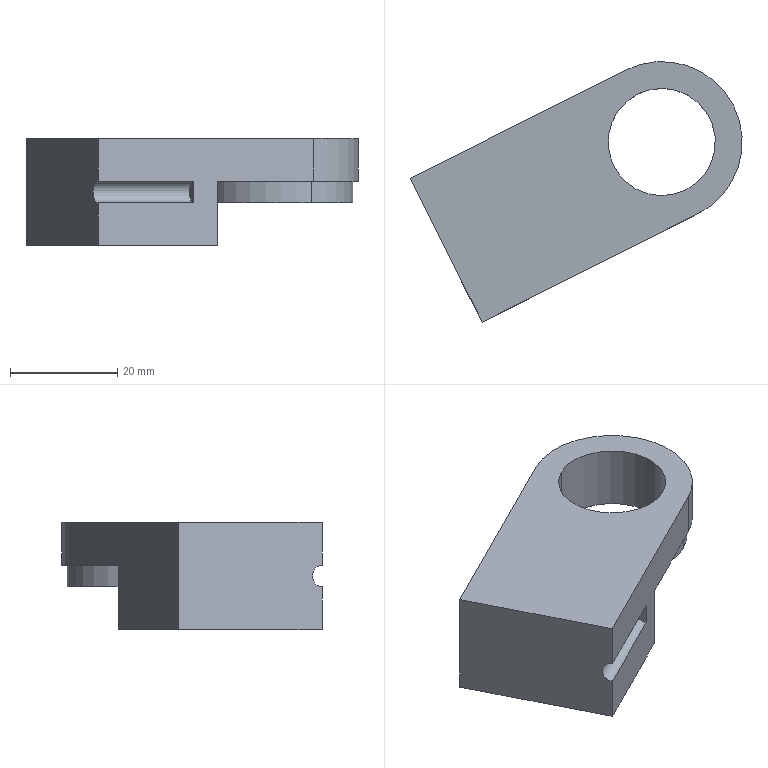Component | SolidWorks | SwingAssistFrame(Left)-2 | 1 solid | 18 faces | box 61.95 x 48.58 x 20 mm | volume 20409 mm3 | plane 10 | cylinder 8 | commonest cylinder face diameters 28 x2 10 x2 20 x2 30 x1 4 x1
build123d program:
from build123d import *

# Parameters (mm, degrees)
SKETCH1_R           = 10
BOSS_EXTRUDE1_DEPTH = 8
SKETCH2_W           = 30
SKETCH2_H           = 25
BOSS_EXTRUDE2_DEPTH = 12
SKETCH5_R           = 2
CUT_EXTRUDE2_DEPTH  = 20
SKETCH10_R          = 5
CUT_EXTRUDE4_DEPTH  = 10
SKETCH6_R           = 14
SKETCH6_R_2         = 10
BOSS_EXTRUDE5_DEPTH = 4


with BuildPart() as part:
    # Sketch1 → Boss-Extrude1 (new body)
    with BuildSketch(Plane.XY):
        with BuildLine():
            Line((-15, 0), (-15, 45))
            Line((-15, 45), (15, 45))
            Line((15, 45), (15, 0))
            ThreePointArc((15, 0), (0, -15), (-15, 0))
        make_face()
        Circle(SKETCH1_R, mode=Mode.SUBTRACT)
    extrude(amount=BOSS_EXTRUDE1_DEPTH)

    # Sketch2 → Boss-Extrude2 (add)
    with BuildSketch(Plane.XY.offset(8)):
        with Locations((0, 32.5)):
            Rectangle(SKETCH2_W, SKETCH2_H)
    extrude(amount=BOSS_EXTRUDE2_DEPTH)

    # Sketch5 → Cut-Extrude2 (cut)
    with BuildSketch(Plane(origin=(0, 45, 0), x_dir=(1, 0, 0), z_dir=(0, 1, 0))):
        with Locations((15, -10)):
            Circle(SKETCH5_R)
    extrude(amount=-CUT_EXTRUDE2_DEPTH, mode=Mode.SUBTRACT)

    # Sketch10 → Cut-Extrude4 (cut)
    with BuildSketch(Plane.XY.offset(20)):
        with Locations((0, 30)):
            Circle(SKETCH10_R)
    extrude(amount=-CUT_EXTRUDE4_DEPTH, mode=Mode.SUBTRACT)

    # Sketch6 → Boss-Extrude5 (add)
    with BuildSketch(Plane.XY.offset(8)):
        Circle(SKETCH6_R)
        Circle(SKETCH6_R_2, mode=Mode.SUBTRACT)
    extrude(amount=BOSS_EXTRUDE5_DEPTH)


solid = part.part

# Placed as in the assembly
solid = solid.moved(Location((17.47, 39.391, 136.846), (180, 0, 63.377)))
STEP:
#1=COLOUR_RGB('',0.7922,0.8196,0.9333);
#2=FILL_AREA_STYLE_COLOUR('',#1);
#3=FILL_AREA_STYLE('',(#2));
#4=SURFACE_STYLE_FILL_AREA(#3);
#5=SURFACE_SIDE_STYLE('',(#4));
#6=SURFACE_STYLE_USAGE(.BOTH.,#5);
#7=PRESENTATION_STYLE_ASSIGNMENT((#6));
#8=CARTESIAN_POINT('',(0.9348,1.058,4.915));
#9=VERTEX_POINT('',#8);
#10=CARTESIAN_POINT('',(0.4408,2.044,4.915));
#11=VERTEX_POINT('',#10);
#12=CARTESIAN_POINT('',(0.6878,1.551,4.915));
#13=DIRECTION('',(0.,0.,-1.));
#14=DIRECTION('',(0.4481,-0.894,0.));
#15=AXIS2_PLACEMENT_3D('',#12,#13,#14);
#16=CIRCLE('',#15,0.5512);
#17=EDGE_CURVE('',#9,#11,#16,.T.);
#18=ORIENTED_EDGE('',*,*,#17,.F.);
#19=CARTESIAN_POINT('',(0.9348,1.058,5.073));
#20=VERTEX_POINT('',#19);
#21=CARTESIAN_POINT('',(0.9348,1.058,4.915));
#22=DIRECTION('',(-0.,-0.,1.));
#23=VECTOR('',#22,39.37);
#24=LINE('',#21,#23);
#25=EDGE_CURVE('',#9,#20,#24,.T.);
#26=ORIENTED_EDGE('',*,*,#25,.T.);
#27=CARTESIAN_POINT('',(0.4408,2.044,5.073));
#28=VERTEX_POINT('',#27);
#29=CARTESIAN_POINT('',(0.6878,1.551,5.073));
#30=DIRECTION('',(0.,0.,-1.));
#31=DIRECTION('',(0.4481,-0.894,0.));
#32=AXIS2_PLACEMENT_3D('',#29,#30,#31);
#33=CIRCLE('',#32,0.5512);
#34=EDGE_CURVE('',#20,#28,#33,.T.);
#35=ORIENTED_EDGE('',*,*,#34,.T.);
#36=CARTESIAN_POINT('',(0.4408,2.044,4.915));
#37=DIRECTION('',(-0.,-0.,1.));
#38=VECTOR('',#37,39.37);
#39=LINE('',#36,#38);
#40=EDGE_CURVE('',#11,#28,#39,.T.);
#41=ORIENTED_EDGE('',*,*,#40,.F.);
#42=EDGE_LOOP('',(#18,#26,#35,#41));
#43=FACE_OUTER_BOUND('',#42,.T.);
#44=CARTESIAN_POINT('',(0.6878,1.551,4.915));
#45=DIRECTION('',(-0.,-0.,1.));
#46=DIRECTION('',(-0.4481,0.894,0.));
#47=AXIS2_PLACEMENT_3D('',#44,#45,#46);
#48=CYLINDRICAL_SURFACE('',#47,0.5512);
#49=ADVANCED_FACE('',(#43),#48,.T.);
#50=CARTESIAN_POINT('',(-0.4563,1.198,4.994));
#51=VERTEX_POINT('',#50);
#52=CARTESIAN_POINT('',(-0.2799,0.8456,4.994));
#53=VERTEX_POINT('',#52);
#54=CARTESIAN_POINT('',(-0.3681,1.022,4.994));
#55=DIRECTION('',(0.,0.,-1.));
#56=DIRECTION('',(0.4481,-0.894,0.));
#57=AXIS2_PLACEMENT_3D('',#54,#55,#56);
#58=CIRCLE('',#57,0.1969);
#59=EDGE_CURVE('',#51,#53,#58,.T.);
#60=ORIENTED_EDGE('',*,*,#59,.F.);
#61=CARTESIAN_POINT('',(-0.4563,1.198,4.6));
#62=VERTEX_POINT('',#61);
#63=CARTESIAN_POINT('',(-0.4563,1.198,4.994));
#64=DIRECTION('',(0.,0.,-1.));
#65=VECTOR('',#64,39.37);
#66=LINE('',#63,#65);
#67=EDGE_CURVE('',#51,#62,#66,.T.);
#68=ORIENTED_EDGE('',*,*,#67,.T.);
#69=CARTESIAN_POINT('',(-0.2799,0.8456,4.6));
#70=VERTEX_POINT('',#69);
#71=CARTESIAN_POINT('',(-0.3681,1.022,4.6));
#72=DIRECTION('',(0.,0.,-1.));
#73=DIRECTION('',(0.4481,-0.894,0.));
#74=AXIS2_PLACEMENT_3D('',#71,#72,#73);
#75=CIRCLE('',#74,0.1969);
#76=EDGE_CURVE('',#62,#70,#75,.T.);
#77=ORIENTED_EDGE('',*,*,#76,.T.);
#78=CARTESIAN_POINT('',(-0.2799,0.8456,4.994));
#79=DIRECTION('',(0.,0.,-1.));
#80=VECTOR('',#79,39.37);
#81=LINE('',#78,#80);
#82=EDGE_CURVE('',#53,#70,#81,.T.);
#83=ORIENTED_EDGE('',*,*,#82,.F.);
#84=EDGE_LOOP('',(#60,#68,#77,#83));
#85=FACE_OUTER_BOUND('',#84,.T.);
#86=CARTESIAN_POINT('',(-0.3681,1.022,4.994));
#87=DIRECTION('',(0.,0.,-1.));
#88=DIRECTION('',(0.4481,-0.894,0.));
#89=AXIS2_PLACEMENT_3D('',#86,#87,#88);
#90=CYLINDRICAL_SURFACE('',#89,0.1969);
#91=ADVANCED_FACE('',(#85),#90,.F.);
#92=CARTESIAN_POINT('',(0.5114,1.903,4.915));
#93=VERTEX_POINT('',#92);
#94=CARTESIAN_POINT('',(0.8642,1.199,4.915));
#95=VERTEX_POINT('',#94);
#96=CARTESIAN_POINT('',(0.6878,1.551,4.915));
#97=DIRECTION('',(0.,0.,-1.));
#98=DIRECTION('',(0.4481,-0.894,0.));
#99=AXIS2_PLACEMENT_3D('',#96,#97,#98);
#100=CIRCLE('',#99,0.3937);
#101=EDGE_CURVE('',#93,#95,#100,.T.);
#102=ORIENTED_EDGE('',*,*,#101,.T.);
#103=CARTESIAN_POINT('',(0.8642,1.199,5.388));
#104=VERTEX_POINT('',#103);
#105=CARTESIAN_POINT('',(0.8642,1.199,5.073));
#106=DIRECTION('',(-0.,-0.,1.));
#107=VECTOR('',#106,39.37);
#108=LINE('',#105,#107);
#109=EDGE_CURVE('',#95,#104,#108,.T.);
#110=ORIENTED_EDGE('',*,*,#109,.T.);
#111=CARTESIAN_POINT('',(0.5114,1.903,5.388));
#112=VERTEX_POINT('',#111);
#113=CARTESIAN_POINT('',(0.6878,1.551,5.388));
#114=DIRECTION('',(0.,0.,-1.));
#115=DIRECTION('',(0.4481,-0.894,0.));
#116=AXIS2_PLACEMENT_3D('',#113,#114,#115);
#117=CIRCLE('',#116,0.3937);
#118=EDGE_CURVE('',#112,#104,#117,.T.);
#119=ORIENTED_EDGE('',*,*,#118,.F.);
#120=CARTESIAN_POINT('',(0.5114,1.903,5.073));
#121=DIRECTION('',(-0.,-0.,1.));
#122=VECTOR('',#121,39.37);
#123=LINE('',#120,#122);
#124=EDGE_CURVE('',#93,#112,#123,.T.);
#125=ORIENTED_EDGE('',*,*,#124,.F.);
#126=EDGE_LOOP('',(#102,#110,#119,#125));
#127=FACE_OUTER_BOUND('',#126,.T.);
#128=CARTESIAN_POINT('',(0.6878,1.551,5.073));
#129=DIRECTION('',(-0.,-0.,1.));
#130=DIRECTION('',(-0.4481,0.894,0.));
#131=AXIS2_PLACEMENT_3D('',#128,#129,#130);
#132=CYLINDRICAL_SURFACE('',#131,0.3937);
#133=ADVANCED_FACE('',(#127),#132,.F.);
#134=CARTESIAN_POINT('',(-0.2808,1.726,5.073));
#135=VERTEX_POINT('',#134);
#136=CARTESIAN_POINT('',(0.2485,0.67,5.073));
#137=VERTEX_POINT('',#136);
#138=CARTESIAN_POINT('',(-0.2808,1.726,5.073));
#139=DIRECTION('',(0.4481,-0.894,-0.));
#140=VECTOR('',#139,39.37);
#141=LINE('',#138,#140);
#142=EDGE_CURVE('',#135,#137,#141,.T.);
#143=ORIENTED_EDGE('',*,*,#142,.F.);
#144=CARTESIAN_POINT('',(0.4231,2.079,5.073));
#145=VERTEX_POINT('',#144);
#146=CARTESIAN_POINT('',(0.4231,2.079,5.073));
#147=DIRECTION('',(0.894,0.4481,0.));
#148=VECTOR('',#147,39.37);
#149=LINE('',#146,#148);
#150=EDGE_CURVE('',#135,#145,#149,.T.);
#151=ORIENTED_EDGE('',*,*,#150,.T.);
#152=CARTESIAN_POINT('',(0.9524,1.023,5.073));
#153=VERTEX_POINT('',#152);
#154=CARTESIAN_POINT('',(0.6878,1.551,5.073));
#155=DIRECTION('',(0.,0.,-1.));
#156=DIRECTION('',(0.4481,-0.894,0.));
#157=AXIS2_PLACEMENT_3D('',#154,#155,#156);
#158=CIRCLE('',#157,0.5906);
#159=EDGE_CURVE('',#145,#153,#158,.T.);
#160=ORIENTED_EDGE('',*,*,#159,.T.);
#161=CARTESIAN_POINT('',(0.9524,1.023,5.073));
#162=DIRECTION('',(-0.894,-0.4481,-0.));
#163=VECTOR('',#162,39.37);
#164=LINE('',#161,#163);
#165=EDGE_CURVE('',#153,#137,#164,.T.);
#166=ORIENTED_EDGE('',*,*,#165,.T.);
#167=EDGE_LOOP('',(#143,#151,#160,#166));
#168=FACE_OUTER_BOUND('',#167,.T.);
#169=CARTESIAN_POINT('',(0.6878,1.551,5.073));
#170=DIRECTION('',(0.,0.,-1.));
#171=DIRECTION('',(0.4481,-0.894,0.));
#172=AXIS2_PLACEMENT_3D('',#169,#170,#171);
#173=CIRCLE('',#172,0.5512);
#174=EDGE_CURVE('',#28,#20,#173,.T.);
#175=ORIENTED_EDGE('',*,*,#174,.F.);
#176=ORIENTED_EDGE('',*,*,#34,.F.);
#177=EDGE_LOOP('',(#175,#176));
#178=FACE_BOUND('',#177,.T.);
#179=CARTESIAN_POINT('',(0.6878,1.551,5.073));
#180=DIRECTION('',(-0.,0.,-1.));
#181=DIRECTION('',(0.4481,-0.894,-0.));
#182=AXIS2_PLACEMENT_3D('',#179,#180,#181);
#183=PLANE('',#182);
#184=ADVANCED_FACE('',(#168,#178),#183,.T.);
#185=CARTESIAN_POINT('',(0.4231,2.079,5.388));
#186=VERTEX_POINT('',#185);
#187=CARTESIAN_POINT('',(0.9524,1.023,5.388));
#188=VERTEX_POINT('',#187);
#189=CARTESIAN_POINT('',(0.6878,1.551,5.388));
#190=DIRECTION('',(0.,0.,-1.));
#191=DIRECTION('',(0.4481,-0.894,0.));
#192=AXIS2_PLACEMENT_3D('',#189,#190,#191);
#193=CIRCLE('',#192,0.5906);
#194=EDGE_CURVE('',#186,#188,#193,.T.);
#195=ORIENTED_EDGE('',*,*,#194,.F.);
#196=CARTESIAN_POINT('',(-1.161,1.285,5.388));
#197=VERTEX_POINT('',#196);
#198=CARTESIAN_POINT('',(0.4231,2.079,5.388));
#199=DIRECTION('',(0.894,0.4481,0.));
#200=VECTOR('',#199,39.37);
#201=LINE('',#198,#200);
#202=EDGE_CURVE('',#197,#186,#201,.T.);
#203=ORIENTED_EDGE('',*,*,#202,.F.);
#204=CARTESIAN_POINT('',(-0.6314,0.229,5.388));
#205=VERTEX_POINT('',#204);
#206=CARTESIAN_POINT('',(-1.161,1.285,5.388));
#207=DIRECTION('',(-0.4481,0.894,0.));
#208=VECTOR('',#207,39.37);
#209=LINE('',#206,#208);
#210=EDGE_CURVE('',#205,#197,#209,.T.);
#211=ORIENTED_EDGE('',*,*,#210,.F.);
#212=CARTESIAN_POINT('',(0.9524,1.023,5.388));
#213=DIRECTION('',(-0.894,-0.4481,-0.));
#214=VECTOR('',#213,39.37);
#215=LINE('',#212,#214);
#216=EDGE_CURVE('',#188,#205,#215,.T.);
#217=ORIENTED_EDGE('',*,*,#216,.F.);
#218=EDGE_LOOP('',(#195,#203,#211,#217));
#219=FACE_OUTER_BOUND('',#218,.T.);
#220=ORIENTED_EDGE('',*,*,#118,.T.);
#221=CARTESIAN_POINT('',(0.6878,1.551,5.388));
#222=DIRECTION('',(0.,0.,-1.));
#223=DIRECTION('',(0.4481,-0.894,0.));
#224=AXIS2_PLACEMENT_3D('',#221,#222,#223);
#225=CIRCLE('',#224,0.3937);
#226=EDGE_CURVE('',#104,#112,#225,.T.);
#227=ORIENTED_EDGE('',*,*,#226,.T.);
#228=EDGE_LOOP('',(#220,#227));
#229=FACE_BOUND('',#228,.T.);
#230=CARTESIAN_POINT('',(0.6878,1.551,5.388));
#231=DIRECTION('',(-0.,0.,-1.));
#232=DIRECTION('',(0.4481,-0.894,-0.));
#233=AXIS2_PLACEMENT_3D('',#230,#231,#232);
#234=PLANE('',#233);
#235=ADVANCED_FACE('',(#219,#229),#234,.F.);
#236=ORIENTED_EDGE('',*,*,#194,.T.);
#237=CARTESIAN_POINT('',(0.9524,1.023,5.073));
#238=DIRECTION('',(-0.,-0.,1.));
#239=VECTOR('',#238,39.37);
#240=LINE('',#237,#239);
#241=EDGE_CURVE('',#153,#188,#240,.T.);
#242=ORIENTED_EDGE('',*,*,#241,.F.);
#243=ORIENTED_EDGE('',*,*,#159,.F.);
#244=CARTESIAN_POINT('',(0.4231,2.079,5.073));
#245=DIRECTION('',(-0.,-0.,1.));
#246=VECTOR('',#245,39.37);
#247=LINE('',#244,#246);
#248=EDGE_CURVE('',#145,#186,#247,.T.);
#249=ORIENTED_EDGE('',*,*,#248,.T.);
#250=EDGE_LOOP('',(#236,#242,#243,#249));
#251=FACE_OUTER_BOUND('',#250,.T.);
#252=CARTESIAN_POINT('',(0.6878,1.551,5.073));
#253=DIRECTION('',(-0.,-0.,1.));
#254=DIRECTION('',(-0.4481,0.894,0.));
#255=AXIS2_PLACEMENT_3D('',#252,#253,#254);
#256=CYLINDRICAL_SURFACE('',#255,0.5906);
#257=ADVANCED_FACE('',(#251),#256,.T.);
#258=CARTESIAN_POINT('',(0.07252,0.5818,4.915));
#259=VERTEX_POINT('',#258);
#260=CARTESIAN_POINT('',(0.07252,0.5818,5.073));
#261=VERTEX_POINT('',#260);
#262=CARTESIAN_POINT('',(0.07252,0.5818,5.073));
#263=DIRECTION('',(-0.,-0.,1.));
#264=VECTOR('',#263,39.37);
#265=LINE('',#262,#264);
#266=EDGE_CURVE('',#259,#261,#265,.T.);
#267=ORIENTED_EDGE('',*,*,#266,.F.);
#268=CARTESIAN_POINT('',(-0.6314,0.229,4.915));
#269=VERTEX_POINT('',#268);
#270=CARTESIAN_POINT('',(0.07252,0.5818,4.915));
#271=DIRECTION('',(-0.894,-0.4481,-0.));
#272=VECTOR('',#271,39.37);
#273=LINE('',#270,#272);
#274=EDGE_CURVE('',#259,#269,#273,.T.);
#275=ORIENTED_EDGE('',*,*,#274,.T.);
#276=CARTESIAN_POINT('',(-0.6314,0.229,4.6));
#277=VERTEX_POINT('',#276);
#278=CARTESIAN_POINT('',(-0.6314,0.229,5.073));
#279=DIRECTION('',(-0.,-0.,1.));
#280=VECTOR('',#279,39.37);
#281=LINE('',#278,#280);
#282=EDGE_CURVE('',#277,#269,#281,.T.);
#283=ORIENTED_EDGE('',*,*,#282,.F.);
#284=CARTESIAN_POINT('',(0.2485,0.67,4.6));
#285=VERTEX_POINT('',#284);
#286=CARTESIAN_POINT('',(0.2485,0.67,4.6));
#287=DIRECTION('',(-0.894,-0.4481,-0.));
#288=VECTOR('',#287,39.37);
#289=LINE('',#286,#288);
#290=EDGE_CURVE('',#285,#277,#289,.T.);
#291=ORIENTED_EDGE('',*,*,#290,.F.);
#292=CARTESIAN_POINT('',(0.2485,0.67,4.6));
#293=DIRECTION('',(-0.,-0.,1.));
#294=VECTOR('',#293,39.37);
#295=LINE('',#292,#294);
#296=EDGE_CURVE('',#285,#137,#295,.T.);
#297=ORIENTED_EDGE('',*,*,#296,.T.);
#298=ORIENTED_EDGE('',*,*,#165,.F.);
#299=ORIENTED_EDGE('',*,*,#241,.T.);
#300=ORIENTED_EDGE('',*,*,#216,.T.);
#301=CARTESIAN_POINT('',(-0.6314,0.229,5.073));
#302=VERTEX_POINT('',#301);
#303=CARTESIAN_POINT('',(-0.6314,0.229,5.073));
#304=DIRECTION('',(-0.,-0.,1.));
#305=VECTOR('',#304,39.37);
#306=LINE('',#303,#305);
#307=EDGE_CURVE('',#302,#205,#306,.T.);
#308=ORIENTED_EDGE('',*,*,#307,.F.);
#309=CARTESIAN_POINT('',(0.07252,0.5818,5.073));
#310=DIRECTION('',(0.894,0.4481,0.));
#311=VECTOR('',#310,39.37);
#312=LINE('',#309,#311);
#313=EDGE_CURVE('',#302,#261,#312,.T.);
#314=ORIENTED_EDGE('',*,*,#313,.T.);
#315=EDGE_LOOP('',(#267,#275,#283,#291,#297,#298,#299,#300,#308,#314));
#316=FACE_OUTER_BOUND('',#315,.T.);
#317=CARTESIAN_POINT('',(0.9524,1.023,5.073));
#318=DIRECTION('',(-0.4481,0.894,0.));
#319=DIRECTION('',(0.,0.,-1.));
#320=AXIS2_PLACEMENT_3D('',#317,#318,#319);
#321=PLANE('',#320);
#322=ADVANCED_FACE('',(#316),#321,.F.);
#323=ORIENTED_EDGE('',*,*,#282,.T.);
#324=CARTESIAN_POINT('',(-0.6314,0.229,4.994));
#325=DIRECTION('',(0.894,0.4481,0.));
#326=DIRECTION('',(0.,-0.,1.));
#327=AXIS2_PLACEMENT_3D('',#324,#325,#326);
#328=CIRCLE('',#327,0.07874);
#329=EDGE_CURVE('',#269,#302,#328,.T.);
#330=ORIENTED_EDGE('',*,*,#329,.T.);
#331=ORIENTED_EDGE('',*,*,#307,.T.);
#332=ORIENTED_EDGE('',*,*,#210,.T.);
#333=CARTESIAN_POINT('',(-1.161,1.285,4.6));
#334=VERTEX_POINT('',#333);
#335=CARTESIAN_POINT('',(-1.161,1.285,5.073));
#336=DIRECTION('',(-0.,-0.,1.));
#337=VECTOR('',#336,39.37);
#338=LINE('',#335,#337);
#339=EDGE_CURVE('',#334,#197,#338,.T.);
#340=ORIENTED_EDGE('',*,*,#339,.F.);
#341=CARTESIAN_POINT('',(-0.6314,0.229,4.6));
#342=DIRECTION('',(-0.4481,0.894,0.));
#343=VECTOR('',#342,39.37);
#344=LINE('',#341,#343);
#345=EDGE_CURVE('',#277,#334,#344,.T.);
#346=ORIENTED_EDGE('',*,*,#345,.F.);
#347=EDGE_LOOP('',(#323,#330,#331,#332,#340,#346));
#348=FACE_OUTER_BOUND('',#347,.T.);
#349=CARTESIAN_POINT('',(-1.161,1.285,5.073));
#350=DIRECTION('',(0.894,0.4481,0.));
#351=DIRECTION('',(-0.,-0.,1.));
#352=AXIS2_PLACEMENT_3D('',#349,#350,#351);
#353=PLANE('',#352);
#354=ADVANCED_FACE('',(#348),#353,.F.);
#355=ORIENTED_EDGE('',*,*,#202,.T.);
#356=ORIENTED_EDGE('',*,*,#248,.F.);
#357=ORIENTED_EDGE('',*,*,#150,.F.);
#358=CARTESIAN_POINT('',(-0.2808,1.726,4.6));
#359=VERTEX_POINT('',#358);
#360=CARTESIAN_POINT('',(-0.2808,1.726,4.6));
#361=DIRECTION('',(-0.,-0.,1.));
#362=VECTOR('',#361,39.37);
#363=LINE('',#360,#362);
#364=EDGE_CURVE('',#359,#135,#363,.T.);
#365=ORIENTED_EDGE('',*,*,#364,.F.);
#366=CARTESIAN_POINT('',(-1.161,1.285,4.6));
#367=DIRECTION('',(0.894,0.4481,0.));
#368=VECTOR('',#367,39.37);
#369=LINE('',#366,#368);
#370=EDGE_CURVE('',#334,#359,#369,.T.);
#371=ORIENTED_EDGE('',*,*,#370,.F.);
#372=ORIENTED_EDGE('',*,*,#339,.T.);
#373=EDGE_LOOP('',(#355,#356,#357,#365,#371,#372));
#374=FACE_OUTER_BOUND('',#373,.T.);
#375=CARTESIAN_POINT('',(0.4231,2.079,5.073));
#376=DIRECTION('',(0.4481,-0.894,-0.));
#377=DIRECTION('',(-0.,-0.,1.));
#378=AXIS2_PLACEMENT_3D('',#375,#376,#377);
#379=PLANE('',#378);
#380=ADVANCED_FACE('',(#374),#379,.F.);
#381=ORIENTED_EDGE('',*,*,#109,.F.);
#382=CARTESIAN_POINT('',(0.6878,1.551,4.915));
#383=DIRECTION('',(0.,0.,-1.));
#384=DIRECTION('',(0.4481,-0.894,0.));
#385=AXIS2_PLACEMENT_3D('',#382,#383,#384);
#386=CIRCLE('',#385,0.3937);
#387=EDGE_CURVE('',#95,#93,#386,.T.);
#388=ORIENTED_EDGE('',*,*,#387,.T.);
#389=ORIENTED_EDGE('',*,*,#124,.T.);
#390=ORIENTED_EDGE('',*,*,#226,.F.);
#391=EDGE_LOOP('',(#381,#388,#389,#390));
#392=FACE_OUTER_BOUND('',#391,.T.);
#393=CARTESIAN_POINT('',(0.6878,1.551,5.073));
#394=DIRECTION('',(-0.,-0.,1.));
#395=DIRECTION('',(-0.4481,0.894,0.));
#396=AXIS2_PLACEMENT_3D('',#393,#394,#395);
#397=CYLINDRICAL_SURFACE('',#396,0.3937);
#398=ADVANCED_FACE('',(#392),#397,.F.);
#399=ORIENTED_EDGE('',*,*,#142,.T.);
#400=ORIENTED_EDGE('',*,*,#296,.F.);
#401=CARTESIAN_POINT('',(-0.2808,1.726,4.6));
#402=DIRECTION('',(0.4481,-0.894,-0.));
#403=VECTOR('',#402,39.37);
#404=LINE('',#401,#403);
#405=EDGE_CURVE('',#359,#285,#404,.T.);
#406=ORIENTED_EDGE('',*,*,#405,.F.);
#407=ORIENTED_EDGE('',*,*,#364,.T.);
#408=EDGE_LOOP('',(#399,#400,#406,#407));
#409=FACE_OUTER_BOUND('',#408,.T.);
#410=CARTESIAN_POINT('',(-0.2808,1.726,4.6));
#411=DIRECTION('',(-0.894,-0.4481,-0.));
#412=DIRECTION('',(0.,0.,-1.));
#413=AXIS2_PLACEMENT_3D('',#410,#411,#412);
#414=PLANE('',#413);
#415=ADVANCED_FACE('',(#409),#414,.F.);
#416=CARTESIAN_POINT('',(-0.3681,1.022,4.6));
#417=DIRECTION('',(0.,0.,-1.));
#418=DIRECTION('',(0.4481,-0.894,0.));
#419=AXIS2_PLACEMENT_3D('',#416,#417,#418);
#420=CIRCLE('',#419,0.1969);
#421=EDGE_CURVE('',#70,#62,#420,.T.);
#422=ORIENTED_EDGE('',*,*,#421,.F.);
#423=ORIENTED_EDGE('',*,*,#76,.F.);
#424=EDGE_LOOP('',(#422,#423));
#425=FACE_BOUND('',#424,.T.);
#426=ORIENTED_EDGE('',*,*,#345,.T.);
#427=ORIENTED_EDGE('',*,*,#370,.T.);
#428=ORIENTED_EDGE('',*,*,#405,.T.);
#429=ORIENTED_EDGE('',*,*,#290,.T.);
#430=EDGE_LOOP('',(#426,#427,#428,#429));
#431=FACE_OUTER_BOUND('',#430,.T.);
#432=CARTESIAN_POINT('',(0.6878,1.551,4.6));
#433=DIRECTION('',(-0.,0.,-1.));
#434=DIRECTION('',(0.4481,-0.894,-0.));
#435=AXIS2_PLACEMENT_3D('',#432,#433,#434);
#436=PLANE('',#435);
#437=ADVANCED_FACE('',(#425,#431),#436,.T.);
#438=ORIENTED_EDGE('',*,*,#266,.T.);
#439=CARTESIAN_POINT('',(0.07252,0.5818,4.994));
#440=DIRECTION('',(-0.894,-0.4481,-0.));
#441=DIRECTION('',(0.,0.,-1.));
#442=AXIS2_PLACEMENT_3D('',#439,#440,#441);
#443=CIRCLE('',#442,0.07874);
#444=EDGE_CURVE('',#261,#259,#443,.T.);
#445=ORIENTED_EDGE('',*,*,#444,.T.);
#446=EDGE_LOOP('',(#438,#445));
#447=FACE_OUTER_BOUND('',#446,.T.);
#448=CARTESIAN_POINT('',(0.07252,0.5818,4.994));
#449=DIRECTION('',(-0.894,-0.4481,-0.));
#450=DIRECTION('',(0.,0.,-1.));
#451=AXIS2_PLACEMENT_3D('',#448,#449,#450);
#452=PLANE('',#451);
#453=ADVANCED_FACE('',(#447),#452,.T.);
#454=ORIENTED_EDGE('',*,*,#444,.F.);
#455=ORIENTED_EDGE('',*,*,#313,.F.);
#456=ORIENTED_EDGE('',*,*,#329,.F.);
#457=ORIENTED_EDGE('',*,*,#274,.F.);
#458=EDGE_LOOP('',(#454,#455,#456,#457));
#459=FACE_OUTER_BOUND('',#458,.T.);
#460=CARTESIAN_POINT('',(0.07252,0.5818,4.994));
#461=DIRECTION('',(-0.894,-0.4481,-0.));
#462=DIRECTION('',(0.,0.,-1.));
#463=AXIS2_PLACEMENT_3D('',#460,#461,#462);
#464=CYLINDRICAL_SURFACE('',#463,0.07874);
#465=ADVANCED_FACE('',(#459),#464,.F.);
#466=ORIENTED_EDGE('',*,*,#67,.F.);
#467=CARTESIAN_POINT('',(-0.3681,1.022,4.994));
#468=DIRECTION('',(0.,0.,-1.));
#469=DIRECTION('',(0.4481,-0.894,0.));
#470=AXIS2_PLACEMENT_3D('',#467,#468,#469);
#471=CIRCLE('',#470,0.1969);
#472=EDGE_CURVE('',#53,#51,#471,.T.);
#473=ORIENTED_EDGE('',*,*,#472,.F.);
#474=ORIENTED_EDGE('',*,*,#82,.T.);
#475=ORIENTED_EDGE('',*,*,#421,.T.);
#476=EDGE_LOOP('',(#466,#473,#474,#475));
#477=FACE_OUTER_BOUND('',#476,.T.);
#478=CARTESIAN_POINT('',(-0.3681,1.022,4.994));
#479=DIRECTION('',(0.,0.,-1.));
#480=DIRECTION('',(0.4481,-0.894,0.));
#481=AXIS2_PLACEMENT_3D('',#478,#479,#480);
#482=CYLINDRICAL_SURFACE('',#481,0.1969);
#483=ADVANCED_FACE('',(#477),#482,.F.);
#484=ORIENTED_EDGE('',*,*,#472,.T.);
#485=ORIENTED_EDGE('',*,*,#59,.T.);
#486=EDGE_LOOP('',(#484,#485));
#487=FACE_OUTER_BOUND('',#486,.T.);
#488=CARTESIAN_POINT('',(-0.3681,1.022,4.994));
#489=DIRECTION('',(-0.,0.,-1.));
#490=DIRECTION('',(0.4481,-0.894,-0.));
#491=AXIS2_PLACEMENT_3D('',#488,#489,#490);
#492=PLANE('',#491);
#493=ADVANCED_FACE('',(#487),#492,.T.);
#494=CARTESIAN_POINT('',(0.6878,1.551,4.915));
#495=DIRECTION('',(0.,0.,-1.));
#496=DIRECTION('',(0.4481,-0.894,0.));
#497=AXIS2_PLACEMENT_3D('',#494,#495,#496);
#498=CIRCLE('',#497,0.5512);
#499=EDGE_CURVE('',#11,#9,#498,.T.);
#500=ORIENTED_EDGE('',*,*,#499,.T.);
#501=ORIENTED_EDGE('',*,*,#17,.T.);
#502=EDGE_LOOP('',(#500,#501));
#503=FACE_OUTER_BOUND('',#502,.T.);
#504=ORIENTED_EDGE('',*,*,#101,.F.);
#505=ORIENTED_EDGE('',*,*,#387,.F.);
#506=EDGE_LOOP('',(#504,#505));
#507=FACE_BOUND('',#506,.T.);
#508=CARTESIAN_POINT('',(0.6878,1.551,4.915));
#509=DIRECTION('',(-0.,0.,-1.));
#510=DIRECTION('',(0.4481,-0.894,-0.));
#511=AXIS2_PLACEMENT_3D('',#508,#509,#510);
#512=PLANE('',#511);
#513=ADVANCED_FACE('',(#503,#507),#512,.T.);
#514=ORIENTED_EDGE('',*,*,#25,.F.);
#515=ORIENTED_EDGE('',*,*,#499,.F.);
#516=ORIENTED_EDGE('',*,*,#40,.T.);
#517=ORIENTED_EDGE('',*,*,#174,.T.);
#518=EDGE_LOOP('',(#514,#515,#516,#517));
#519=FACE_OUTER_BOUND('',#518,.T.);
#520=CARTESIAN_POINT('',(0.6878,1.551,4.915));
#521=DIRECTION('',(-0.,-0.,1.));
#522=DIRECTION('',(-0.4481,0.894,0.));
#523=AXIS2_PLACEMENT_3D('',#520,#521,#522);
#524=CYLINDRICAL_SURFACE('',#523,0.5512);
#525=ADVANCED_FACE('',(#519),#524,.T.);
#526=CLOSED_SHELL('',(#49,#91,#133,#184,#235,#257,#322,#354,#380,#398,#415,#437,#453,#465,#483,#493,#513,#525));
#527=MANIFOLD_SOLID_BREP('',#526);
#528=STYLED_ITEM('',(#7),#527);
#529=PRESENTATION_LAYER_ASSIGNMENT('','',(#528));
#530=CARTESIAN_POINT('',(0.,0.,0.));
#531=DIRECTION('',(0.,0.,1.));
#532=DIRECTION('',(1.,0.,0.));
#533=AXIS2_PLACEMENT_3D('',#530,#531,#532);
#534=(LENGTH_UNIT()NAMED_UNIT(*)SI_UNIT($,.METRE.));
#535=LENGTH_MEASURE_WITH_UNIT(LENGTH_MEASURE(0.0254),#534);
#536=DIMENSIONAL_EXPONENTS(1.,0.,0.,0.,0.,0.,0.);
#537=(CONVERSION_BASED_UNIT('',#535)LENGTH_UNIT()NAMED_UNIT(#536));
#538=UNCERTAINTY_MEASURE_WITH_UNIT(LENGTH_MEASURE(0.00001),#537,'','');
#539=(NAMED_UNIT(*)PLANE_ANGLE_UNIT()SI_UNIT($,.RADIAN.));
#540=(NAMED_UNIT(*)SI_UNIT($,.STERADIAN.)SOLID_ANGLE_UNIT());
#541=(GEOMETRIC_REPRESENTATION_CONTEXT(3)GLOBAL_UNCERTAINTY_ASSIGNED_CONTEXT((#538))GLOBAL_UNIT_ASSIGNED_CONTEXT((#537,#539,#540))REPRESENTATION_CONTEXT('',''));
#542=ADVANCED_BREP_SHAPE_REPRESENTATION('',(#527,#533),#541);
#543=(LENGTH_UNIT()NAMED_UNIT(*)SI_UNIT($,.METRE.));
#544=LENGTH_MEASURE_WITH_UNIT(LENGTH_MEASURE(0.0254),#543);
#545=DIMENSIONAL_EXPONENTS(1.,0.,0.,0.,0.,0.,0.);
#546=(CONVERSION_BASED_UNIT('',#544)LENGTH_UNIT()NAMED_UNIT(#545));
#547=UNCERTAINTY_MEASURE_WITH_UNIT(LENGTH_MEASURE(0.00001),#546,'','');
#548=(NAMED_UNIT(*)PLANE_ANGLE_UNIT()SI_UNIT($,.RADIAN.));
#549=(NAMED_UNIT(*)SI_UNIT($,.STERADIAN.)SOLID_ANGLE_UNIT());
#550=(GEOMETRIC_REPRESENTATION_CONTEXT(3)GLOBAL_UNCERTAINTY_ASSIGNED_CONTEXT((#547))GLOBAL_UNIT_ASSIGNED_CONTEXT((#546,#548,#549))REPRESENTATION_CONTEXT('',''));
#551=MECHANICAL_DESIGN_GEOMETRIC_PRESENTATION_REPRESENTATION('',(#528),#550);